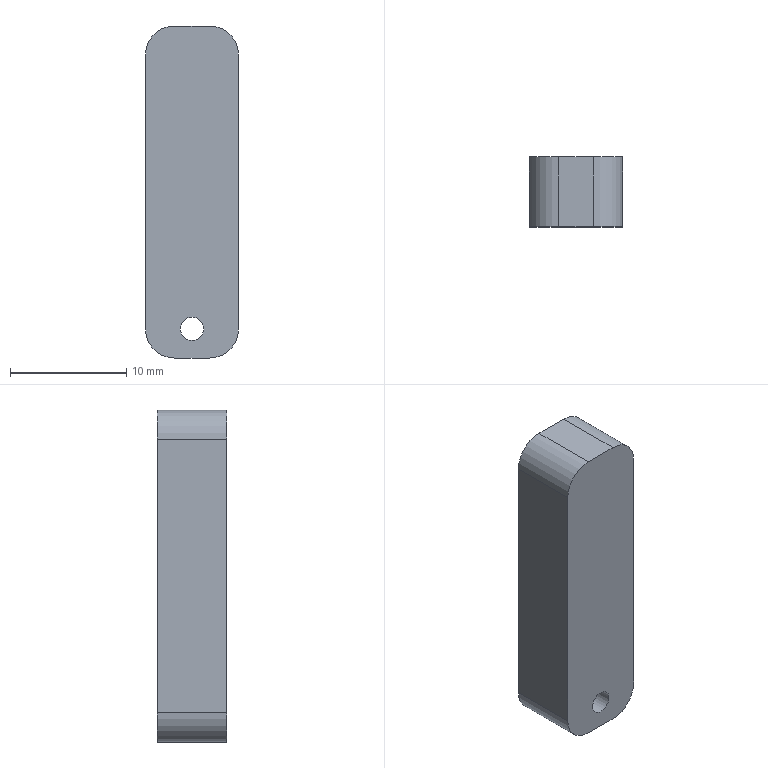Component | NX | ROBOT_ARM_SHORT_ARM | 1 solid | 11 faces | box 8 x 6 x 28.5 mm | volume 1317 mm3 | plane 6 | cylinder 5 | commonest cylinder face diameters 5 x4 2 x1
STEP:
#1=CARTESIAN_POINT('',(0.,0.,0.));
#2=DIRECTION('',(0.,0.,1.));
#3=DIRECTION('',(1.,0.,0.));
#4=AXIS2_PLACEMENT_3D('',#1,#2,#3);
#5=CARTESIAN_POINT('',(7.471,11.498,87.674));
#6=VERTEX_POINT('',#5);
#7=CARTESIAN_POINT('',(7.471,11.498,111.174));
#8=VERTEX_POINT('',#7);
#9=CARTESIAN_POINT('',(7.471,11.498,87.674));
#10=DIRECTION('',(0.,0.,1.));
#11=VECTOR('',#10,1.);
#12=LINE('',#9,#11);
#13=CARTESIAN_POINT('',(7.471,17.498,87.674));
#14=DIRECTION('',(1.,0.,-0.));
#15=DIRECTION('',(-0.,0.,-1.));
#16=AXIS2_PLACEMENT_3D('',#13,#14,#15);
#17=PLANE('',#16);
#18=CARTESIAN_POINT('',(0.,-6.));
#19=DIRECTION('',(-1.,0.));
#20=VECTOR('',#19,1.);
#21=LINE('',#18,#20);
#22=(GEOMETRIC_REPRESENTATION_CONTEXT(2)PARAMETRIC_REPRESENTATION_CONTEXT()REPRESENTATION_CONTEXT('',''));
#23=DEFINITIONAL_REPRESENTATION('',(#21),#22);
#24=PCURVE('',#17,#23);
#25=CARTESIAN_POINT('',(9.971,11.498,111.174));
#26=DIRECTION('',(0.,1.,0.));
#27=DIRECTION('',(1.,0.,0.));
#28=AXIS2_PLACEMENT_3D('',#25,#26,#27);
#29=PLANE('',#28);
#30=CARTESIAN_POINT('',(-2.5,23.5));
#31=DIRECTION('',(0.,-1.));
#32=VECTOR('',#31,1.);
#33=LINE('',#30,#32);
#34=(GEOMETRIC_REPRESENTATION_CONTEXT(2)PARAMETRIC_REPRESENTATION_CONTEXT()REPRESENTATION_CONTEXT('',''));
#35=DEFINITIONAL_REPRESENTATION('',(#33),#34);
#36=PCURVE('',#29,#35);
#37=SURFACE_CURVE('',#12,(#24,#36),.PCURVE_S1.);
#38=EDGE_CURVE('',#6,#8,#37,.T.);
#39=ORIENTED_EDGE('',*,*,#38,.T.);
#40=CARTESIAN_POINT('',(7.471,17.498,111.174));
#41=VERTEX_POINT('',#40);
#42=CARTESIAN_POINT('',(7.471,17.498,111.174));
#43=DIRECTION('',(0.,-1.,0.));
#44=VECTOR('',#43,1.);
#45=LINE('',#42,#44);
#46=CARTESIAN_POINT('',(-23.5,0.));
#47=DIRECTION('',(0.,-1.));
#48=VECTOR('',#47,1.);
#49=LINE('',#46,#48);
#50=(GEOMETRIC_REPRESENTATION_CONTEXT(2)PARAMETRIC_REPRESENTATION_CONTEXT()REPRESENTATION_CONTEXT('',''));
#51=DEFINITIONAL_REPRESENTATION('',(#49),#50);
#52=PCURVE('',#17,#51);
#53=CARTESIAN_POINT('',(9.971,17.498,111.174));
#54=DIRECTION('',(0.,-1.,0.));
#55=DIRECTION('',(-1.,0.,0.));
#56=AXIS2_PLACEMENT_3D('',#53,#54,#55);
#57=CYLINDRICAL_SURFACE('',#56,2.5);
#58=CARTESIAN_POINT('',(6.283,0.));
#59=DIRECTION('',(0.,1.));
#60=VECTOR('',#59,1.);
#61=LINE('',#58,#60);
#62=(GEOMETRIC_REPRESENTATION_CONTEXT(2)PARAMETRIC_REPRESENTATION_CONTEXT()REPRESENTATION_CONTEXT('',''));
#63=DEFINITIONAL_REPRESENTATION('',(#61),#62);
#64=PCURVE('',#57,#63);
#65=SURFACE_CURVE('',#45,(#52,#64),.PCURVE_S1.);
#66=EDGE_CURVE('',#41,#8,#65,.T.);
#67=ORIENTED_EDGE('',*,*,#66,.F.);
#68=CARTESIAN_POINT('',(7.471,17.498,87.674));
#69=VERTEX_POINT('',#68);
#70=CARTESIAN_POINT('',(7.471,17.498,87.674));
#71=DIRECTION('',(0.,0.,1.));
#72=VECTOR('',#71,1.);
#73=LINE('',#70,#72);
#74=CARTESIAN_POINT('',(0.,0.));
#75=DIRECTION('',(-1.,0.));
#76=VECTOR('',#75,1.);
#77=LINE('',#74,#76);
#78=(GEOMETRIC_REPRESENTATION_CONTEXT(2)PARAMETRIC_REPRESENTATION_CONTEXT()REPRESENTATION_CONTEXT('',''));
#79=DEFINITIONAL_REPRESENTATION('',(#77),#78);
#80=PCURVE('',#17,#79);
#81=CARTESIAN_POINT('',(9.971,17.498,111.174));
#82=DIRECTION('',(0.,1.,0.));
#83=DIRECTION('',(1.,0.,0.));
#84=AXIS2_PLACEMENT_3D('',#81,#82,#83);
#85=PLANE('',#84);
#86=CARTESIAN_POINT('',(-2.5,23.5));
#87=DIRECTION('',(0.,-1.));
#88=VECTOR('',#87,1.);
#89=LINE('',#86,#88);
#90=(GEOMETRIC_REPRESENTATION_CONTEXT(2)PARAMETRIC_REPRESENTATION_CONTEXT()REPRESENTATION_CONTEXT('',''));
#91=DEFINITIONAL_REPRESENTATION('',(#89),#90);
#92=PCURVE('',#85,#91);
#93=SURFACE_CURVE('',#73,(#80,#92),.PCURVE_S1.);
#94=EDGE_CURVE('',#69,#41,#93,.T.);
#95=ORIENTED_EDGE('',*,*,#94,.F.);
#96=CARTESIAN_POINT('',(7.471,17.498,87.674));
#97=DIRECTION('',(0.,-1.,0.));
#98=VECTOR('',#97,1.);
#99=LINE('',#96,#98);
#100=CARTESIAN_POINT('',(0.,0.));
#101=DIRECTION('',(0.,-1.));
#102=VECTOR('',#101,1.);
#103=LINE('',#100,#102);
#104=(GEOMETRIC_REPRESENTATION_CONTEXT(2)PARAMETRIC_REPRESENTATION_CONTEXT()REPRESENTATION_CONTEXT('',''));
#105=DEFINITIONAL_REPRESENTATION('',(#103),#104);
#106=PCURVE('',#17,#105);
#107=CARTESIAN_POINT('',(9.971,17.498,87.674));
#108=DIRECTION('',(0.,-1.,0.));
#109=DIRECTION('',(-1.,0.,0.));
#110=AXIS2_PLACEMENT_3D('',#107,#108,#109);
#111=CYLINDRICAL_SURFACE('',#110,2.5);
#112=CARTESIAN_POINT('',(0.,0.));
#113=DIRECTION('',(0.,1.));
#114=VECTOR('',#113,1.);
#115=LINE('',#112,#114);
#116=(GEOMETRIC_REPRESENTATION_CONTEXT(2)PARAMETRIC_REPRESENTATION_CONTEXT()REPRESENTATION_CONTEXT('',''));
#117=DEFINITIONAL_REPRESENTATION('',(#115),#116);
#118=PCURVE('',#111,#117);
#119=SURFACE_CURVE('',#99,(#106,#118),.PCURVE_S1.);
#120=EDGE_CURVE('',#69,#6,#119,.T.);
#121=ORIENTED_EDGE('',*,*,#120,.T.);
#122=EDGE_LOOP('',(#39,#67,#95,#121));
#123=FACE_BOUND('',#122,.T.);
#124=ADVANCED_FACE('',(#123),#17,.F.);
#125=CARTESIAN_POINT('',(9.971,11.498,113.674));
#126=VERTEX_POINT('',#125);
#127=CARTESIAN_POINT('',(9.971,11.498,111.174));
#128=DIRECTION('',(0.,1.,0.));
#129=DIRECTION('',(1.,0.,0.));
#130=AXIS2_PLACEMENT_3D('',#127,#128,#129);
#131=CIRCLE('',#130,2.5);
#132=CARTESIAN_POINT('',(9.425,6.));
#133=DIRECTION('',(-1.,0.));
#134=VECTOR('',#133,1.);
#135=LINE('',#132,#134);
#136=(GEOMETRIC_REPRESENTATION_CONTEXT(2)PARAMETRIC_REPRESENTATION_CONTEXT()REPRESENTATION_CONTEXT('',''));
#137=DEFINITIONAL_REPRESENTATION('',(#135),#136);
#138=PCURVE('',#57,#137);
#139=CARTESIAN_POINT('',(0.,0.));
#140=DIRECTION('',(1.,0.));
#141=AXIS2_PLACEMENT_2D('',#139,#140);
#142=CIRCLE('',#141,2.5);
#143=(GEOMETRIC_REPRESENTATION_CONTEXT(2)PARAMETRIC_REPRESENTATION_CONTEXT()REPRESENTATION_CONTEXT('',''));
#144=DEFINITIONAL_REPRESENTATION('',(#142),#143);
#145=PCURVE('',#29,#144);
#146=SURFACE_CURVE('',#131,(#138,#145),.PCURVE_S1.);
#147=EDGE_CURVE('',#8,#126,#146,.T.);
#148=ORIENTED_EDGE('',*,*,#147,.T.);
#149=CARTESIAN_POINT('',(9.971,17.498,113.674));
#150=VERTEX_POINT('',#149);
#151=CARTESIAN_POINT('',(9.971,17.498,113.674));
#152=DIRECTION('',(0.,-1.,0.));
#153=VECTOR('',#152,1.);
#154=LINE('',#151,#153);
#155=CARTESIAN_POINT('',(4.712,0.));
#156=DIRECTION('',(0.,1.));
#157=VECTOR('',#156,1.);
#158=LINE('',#155,#157);
#159=(GEOMETRIC_REPRESENTATION_CONTEXT(2)PARAMETRIC_REPRESENTATION_CONTEXT()REPRESENTATION_CONTEXT('',''));
#160=DEFINITIONAL_REPRESENTATION('',(#158),#159);
#161=PCURVE('',#57,#160);
#162=CARTESIAN_POINT('',(9.971,17.498,113.674));
#163=DIRECTION('',(-0.,0.,-1.));
#164=DIRECTION('',(-1.,0.,0.));
#165=AXIS2_PLACEMENT_3D('',#162,#163,#164);
#166=PLANE('',#165);
#167=CARTESIAN_POINT('',(0.,0.));
#168=DIRECTION('',(0.,-1.));
#169=VECTOR('',#168,1.);
#170=LINE('',#167,#169);
#171=(GEOMETRIC_REPRESENTATION_CONTEXT(2)PARAMETRIC_REPRESENTATION_CONTEXT()REPRESENTATION_CONTEXT('',''));
#172=DEFINITIONAL_REPRESENTATION('',(#170),#171);
#173=PCURVE('',#166,#172);
#174=SURFACE_CURVE('',#154,(#161,#173),.PCURVE_S1.);
#175=EDGE_CURVE('',#150,#126,#174,.T.);
#176=ORIENTED_EDGE('',*,*,#175,.F.);
#177=CARTESIAN_POINT('',(9.971,17.498,111.174));
#178=DIRECTION('',(0.,1.,0.));
#179=DIRECTION('',(1.,0.,0.));
#180=AXIS2_PLACEMENT_3D('',#177,#178,#179);
#181=CIRCLE('',#180,2.5);
#182=CARTESIAN_POINT('',(9.425,0.));
#183=DIRECTION('',(-1.,0.));
#184=VECTOR('',#183,1.);
#185=LINE('',#182,#184);
#186=(GEOMETRIC_REPRESENTATION_CONTEXT(2)PARAMETRIC_REPRESENTATION_CONTEXT()REPRESENTATION_CONTEXT('',''));
#187=DEFINITIONAL_REPRESENTATION('',(#185),#186);
#188=PCURVE('',#57,#187);
#189=CARTESIAN_POINT('',(0.,0.));
#190=DIRECTION('',(1.,0.));
#191=AXIS2_PLACEMENT_2D('',#189,#190);
#192=CIRCLE('',#191,2.5);
#193=(GEOMETRIC_REPRESENTATION_CONTEXT(2)PARAMETRIC_REPRESENTATION_CONTEXT()REPRESENTATION_CONTEXT('',''));
#194=DEFINITIONAL_REPRESENTATION('',(#192),#193);
#195=PCURVE('',#85,#194);
#196=SURFACE_CURVE('',#181,(#188,#195),.PCURVE_S1.);
#197=EDGE_CURVE('',#41,#150,#196,.T.);
#198=ORIENTED_EDGE('',*,*,#197,.F.);
#199=ORIENTED_EDGE('',*,*,#66,.T.);
#200=EDGE_LOOP('',(#148,#176,#198,#199));
#201=FACE_BOUND('',#200,.T.);
#202=ADVANCED_FACE('',(#201),#57,.T.);
#203=CARTESIAN_POINT('',(12.971,11.498,113.674));
#204=VERTEX_POINT('',#203);
#205=CARTESIAN_POINT('',(9.971,11.498,113.674));
#206=DIRECTION('',(1.,0.,-0.));
#207=VECTOR('',#206,1.);
#208=LINE('',#205,#207);
#209=CARTESIAN_POINT('',(0.,-6.));
#210=DIRECTION('',(-1.,0.));
#211=VECTOR('',#210,1.);
#212=LINE('',#209,#211);
#213=(GEOMETRIC_REPRESENTATION_CONTEXT(2)PARAMETRIC_REPRESENTATION_CONTEXT()REPRESENTATION_CONTEXT('',''));
#214=DEFINITIONAL_REPRESENTATION('',(#212),#213);
#215=PCURVE('',#166,#214);
#216=CARTESIAN_POINT('',(0.,-2.5));
#217=DIRECTION('',(1.,0.));
#218=VECTOR('',#217,1.);
#219=LINE('',#216,#218);
#220=(GEOMETRIC_REPRESENTATION_CONTEXT(2)PARAMETRIC_REPRESENTATION_CONTEXT()REPRESENTATION_CONTEXT('',''));
#221=DEFINITIONAL_REPRESENTATION('',(#219),#220);
#222=PCURVE('',#29,#221);
#223=SURFACE_CURVE('',#208,(#215,#222),.PCURVE_S1.);
#224=EDGE_CURVE('',#126,#204,#223,.T.);
#225=ORIENTED_EDGE('',*,*,#224,.T.);
#226=CARTESIAN_POINT('',(12.971,17.498,113.674));
#227=VERTEX_POINT('',#226);
#228=CARTESIAN_POINT('',(12.971,17.498,113.674));
#229=DIRECTION('',(0.,-1.,0.));
#230=VECTOR('',#229,1.);
#231=LINE('',#228,#230);
#232=CARTESIAN_POINT('',(-3.,0.));
#233=DIRECTION('',(0.,-1.));
#234=VECTOR('',#233,1.);
#235=LINE('',#232,#234);
#236=(GEOMETRIC_REPRESENTATION_CONTEXT(2)PARAMETRIC_REPRESENTATION_CONTEXT()REPRESENTATION_CONTEXT('',''));
#237=DEFINITIONAL_REPRESENTATION('',(#235),#236);
#238=PCURVE('',#166,#237);
#239=CARTESIAN_POINT('',(12.971,17.498,111.174));
#240=DIRECTION('',(0.,-1.,0.));
#241=DIRECTION('',(-1.,0.,0.));
#242=AXIS2_PLACEMENT_3D('',#239,#240,#241);
#243=CYLINDRICAL_SURFACE('',#242,2.5);
#244=CARTESIAN_POINT('',(4.712,0.));
#245=DIRECTION('',(0.,1.));
#246=VECTOR('',#245,1.);
#247=LINE('',#244,#246);
#248=(GEOMETRIC_REPRESENTATION_CONTEXT(2)PARAMETRIC_REPRESENTATION_CONTEXT()REPRESENTATION_CONTEXT('',''));
#249=DEFINITIONAL_REPRESENTATION('',(#247),#248);
#250=PCURVE('',#243,#249);
#251=SURFACE_CURVE('',#231,(#238,#250),.PCURVE_S1.);
#252=EDGE_CURVE('',#227,#204,#251,.T.);
#253=ORIENTED_EDGE('',*,*,#252,.F.);
#254=CARTESIAN_POINT('',(9.971,17.498,113.674));
#255=DIRECTION('',(1.,0.,-0.));
#256=VECTOR('',#255,1.);
#257=LINE('',#254,#256);
#258=CARTESIAN_POINT('',(0.,0.));
#259=DIRECTION('',(-1.,0.));
#260=VECTOR('',#259,1.);
#261=LINE('',#258,#260);
#262=(GEOMETRIC_REPRESENTATION_CONTEXT(2)PARAMETRIC_REPRESENTATION_CONTEXT()REPRESENTATION_CONTEXT('',''));
#263=DEFINITIONAL_REPRESENTATION('',(#261),#262);
#264=PCURVE('',#166,#263);
#265=CARTESIAN_POINT('',(0.,-2.5));
#266=DIRECTION('',(1.,0.));
#267=VECTOR('',#266,1.);
#268=LINE('',#265,#267);
#269=(GEOMETRIC_REPRESENTATION_CONTEXT(2)PARAMETRIC_REPRESENTATION_CONTEXT()REPRESENTATION_CONTEXT('',''));
#270=DEFINITIONAL_REPRESENTATION('',(#268),#269);
#271=PCURVE('',#85,#270);
#272=SURFACE_CURVE('',#257,(#264,#271),.PCURVE_S1.);
#273=EDGE_CURVE('',#150,#227,#272,.T.);
#274=ORIENTED_EDGE('',*,*,#273,.F.);
#275=ORIENTED_EDGE('',*,*,#175,.T.);
#276=EDGE_LOOP('',(#225,#253,#274,#275));
#277=FACE_BOUND('',#276,.T.);
#278=ADVANCED_FACE('',(#277),#166,.F.);
#279=CARTESIAN_POINT('',(15.471,11.498,111.174));
#280=VERTEX_POINT('',#279);
#281=CARTESIAN_POINT('',(12.971,11.498,111.174));
#282=DIRECTION('',(0.,1.,0.));
#283=DIRECTION('',(1.,0.,0.));
#284=AXIS2_PLACEMENT_3D('',#281,#282,#283);
#285=CIRCLE('',#284,2.5);
#286=CARTESIAN_POINT('',(9.425,6.));
#287=DIRECTION('',(-1.,0.));
#288=VECTOR('',#287,1.);
#289=LINE('',#286,#288);
#290=(GEOMETRIC_REPRESENTATION_CONTEXT(2)PARAMETRIC_REPRESENTATION_CONTEXT()REPRESENTATION_CONTEXT('',''));
#291=DEFINITIONAL_REPRESENTATION('',(#289),#290);
#292=PCURVE('',#243,#291);
#293=CARTESIAN_POINT('',(3.,0.));
#294=DIRECTION('',(1.,0.));
#295=AXIS2_PLACEMENT_2D('',#293,#294);
#296=CIRCLE('',#295,2.5);
#297=(GEOMETRIC_REPRESENTATION_CONTEXT(2)PARAMETRIC_REPRESENTATION_CONTEXT()REPRESENTATION_CONTEXT('',''));
#298=DEFINITIONAL_REPRESENTATION('',(#296),#297);
#299=PCURVE('',#29,#298);
#300=SURFACE_CURVE('',#285,(#292,#299),.PCURVE_S1.);
#301=EDGE_CURVE('',#204,#280,#300,.T.);
#302=ORIENTED_EDGE('',*,*,#301,.T.);
#303=CARTESIAN_POINT('',(15.471,17.498,111.174));
#304=VERTEX_POINT('',#303);
#305=CARTESIAN_POINT('',(15.471,17.498,111.174));
#306=DIRECTION('',(0.,-1.,0.));
#307=VECTOR('',#306,1.);
#308=LINE('',#305,#307);
#309=CARTESIAN_POINT('',(3.142,0.));
#310=DIRECTION('',(0.,1.));
#311=VECTOR('',#310,1.);
#312=LINE('',#309,#311);
#313=(GEOMETRIC_REPRESENTATION_CONTEXT(2)PARAMETRIC_REPRESENTATION_CONTEXT()REPRESENTATION_CONTEXT('',''));
#314=DEFINITIONAL_REPRESENTATION('',(#312),#313);
#315=PCURVE('',#243,#314);
#316=CARTESIAN_POINT('',(15.471,17.498,111.174));
#317=DIRECTION('',(-1.,0.,0.));
#318=DIRECTION('',(0.,0.,1.));
#319=AXIS2_PLACEMENT_3D('',#316,#317,#318);
#320=PLANE('',#319);
#321=CARTESIAN_POINT('',(0.,0.));
#322=DIRECTION('',(0.,-1.));
#323=VECTOR('',#322,1.);
#324=LINE('',#321,#323);
#325=(GEOMETRIC_REPRESENTATION_CONTEXT(2)PARAMETRIC_REPRESENTATION_CONTEXT()REPRESENTATION_CONTEXT('',''));
#326=DEFINITIONAL_REPRESENTATION('',(#324),#325);
#327=PCURVE('',#320,#326);
#328=SURFACE_CURVE('',#308,(#315,#327),.PCURVE_S1.);
#329=EDGE_CURVE('',#304,#280,#328,.T.);
#330=ORIENTED_EDGE('',*,*,#329,.F.);
#331=CARTESIAN_POINT('',(12.971,17.498,111.174));
#332=DIRECTION('',(0.,1.,0.));
#333=DIRECTION('',(1.,0.,0.));
#334=AXIS2_PLACEMENT_3D('',#331,#332,#333);
#335=CIRCLE('',#334,2.5);
#336=CARTESIAN_POINT('',(9.425,0.));
#337=DIRECTION('',(-1.,0.));
#338=VECTOR('',#337,1.);
#339=LINE('',#336,#338);
#340=(GEOMETRIC_REPRESENTATION_CONTEXT(2)PARAMETRIC_REPRESENTATION_CONTEXT()REPRESENTATION_CONTEXT('',''));
#341=DEFINITIONAL_REPRESENTATION('',(#339),#340);
#342=PCURVE('',#243,#341);
#343=CARTESIAN_POINT('',(3.,0.));
#344=DIRECTION('',(1.,0.));
#345=AXIS2_PLACEMENT_2D('',#343,#344);
#346=CIRCLE('',#345,2.5);
#347=(GEOMETRIC_REPRESENTATION_CONTEXT(2)PARAMETRIC_REPRESENTATION_CONTEXT()REPRESENTATION_CONTEXT('',''));
#348=DEFINITIONAL_REPRESENTATION('',(#346),#347);
#349=PCURVE('',#85,#348);
#350=SURFACE_CURVE('',#335,(#342,#349),.PCURVE_S1.);
#351=EDGE_CURVE('',#227,#304,#350,.T.);
#352=ORIENTED_EDGE('',*,*,#351,.F.);
#353=ORIENTED_EDGE('',*,*,#252,.T.);
#354=EDGE_LOOP('',(#302,#330,#352,#353));
#355=FACE_BOUND('',#354,.T.);
#356=ADVANCED_FACE('',(#355),#243,.T.);
#357=CARTESIAN_POINT('',(15.471,11.498,87.674));
#358=VERTEX_POINT('',#357);
#359=CARTESIAN_POINT('',(15.471,11.498,111.174));
#360=DIRECTION('',(-0.,0.,-1.));
#361=VECTOR('',#360,1.);
#362=LINE('',#359,#361);
#363=CARTESIAN_POINT('',(0.,-6.));
#364=DIRECTION('',(-1.,0.));
#365=VECTOR('',#364,1.);
#366=LINE('',#363,#365);
#367=(GEOMETRIC_REPRESENTATION_CONTEXT(2)PARAMETRIC_REPRESENTATION_CONTEXT()REPRESENTATION_CONTEXT('',''));
#368=DEFINITIONAL_REPRESENTATION('',(#366),#367);
#369=PCURVE('',#320,#368);
#370=CARTESIAN_POINT('',(5.5,0.));
#371=DIRECTION('',(-0.,1.));
#372=VECTOR('',#371,1.);
#373=LINE('',#370,#372);
#374=(GEOMETRIC_REPRESENTATION_CONTEXT(2)PARAMETRIC_REPRESENTATION_CONTEXT()REPRESENTATION_CONTEXT('',''));
#375=DEFINITIONAL_REPRESENTATION('',(#373),#374);
#376=PCURVE('',#29,#375);
#377=SURFACE_CURVE('',#362,(#369,#376),.PCURVE_S1.);
#378=EDGE_CURVE('',#280,#358,#377,.T.);
#379=ORIENTED_EDGE('',*,*,#378,.T.);
#380=CARTESIAN_POINT('',(15.471,17.498,87.674));
#381=VERTEX_POINT('',#380);
#382=CARTESIAN_POINT('',(15.471,17.498,87.674));
#383=DIRECTION('',(0.,-1.,0.));
#384=VECTOR('',#383,1.);
#385=LINE('',#382,#384);
#386=CARTESIAN_POINT('',(-23.5,0.));
#387=DIRECTION('',(0.,-1.));
#388=VECTOR('',#387,1.);
#389=LINE('',#386,#388);
#390=(GEOMETRIC_REPRESENTATION_CONTEXT(2)PARAMETRIC_REPRESENTATION_CONTEXT()REPRESENTATION_CONTEXT('',''));
#391=DEFINITIONAL_REPRESENTATION('',(#389),#390);
#392=PCURVE('',#320,#391);
#393=CARTESIAN_POINT('',(12.971,17.498,87.674));
#394=DIRECTION('',(0.,-1.,0.));
#395=DIRECTION('',(-1.,0.,0.));
#396=AXIS2_PLACEMENT_3D('',#393,#394,#395);
#397=CYLINDRICAL_SURFACE('',#396,2.5);
#398=CARTESIAN_POINT('',(3.142,0.));
#399=DIRECTION('',(0.,1.));
#400=VECTOR('',#399,1.);
#401=LINE('',#398,#400);
#402=(GEOMETRIC_REPRESENTATION_CONTEXT(2)PARAMETRIC_REPRESENTATION_CONTEXT()REPRESENTATION_CONTEXT('',''));
#403=DEFINITIONAL_REPRESENTATION('',(#401),#402);
#404=PCURVE('',#397,#403);
#405=SURFACE_CURVE('',#385,(#392,#404),.PCURVE_S1.);
#406=EDGE_CURVE('',#381,#358,#405,.T.);
#407=ORIENTED_EDGE('',*,*,#406,.F.);
#408=CARTESIAN_POINT('',(15.471,17.498,111.174));
#409=DIRECTION('',(-0.,0.,-1.));
#410=VECTOR('',#409,1.);
#411=LINE('',#408,#410);
#412=CARTESIAN_POINT('',(0.,0.));
#413=DIRECTION('',(-1.,0.));
#414=VECTOR('',#413,1.);
#415=LINE('',#412,#414);
#416=(GEOMETRIC_REPRESENTATION_CONTEXT(2)PARAMETRIC_REPRESENTATION_CONTEXT()REPRESENTATION_CONTEXT('',''));
#417=DEFINITIONAL_REPRESENTATION('',(#415),#416);
#418=PCURVE('',#320,#417);
#419=CARTESIAN_POINT('',(5.5,0.));
#420=DIRECTION('',(-0.,1.));
#421=VECTOR('',#420,1.);
#422=LINE('',#419,#421);
#423=(GEOMETRIC_REPRESENTATION_CONTEXT(2)PARAMETRIC_REPRESENTATION_CONTEXT()REPRESENTATION_CONTEXT('',''));
#424=DEFINITIONAL_REPRESENTATION('',(#422),#423);
#425=PCURVE('',#85,#424);
#426=SURFACE_CURVE('',#411,(#418,#425),.PCURVE_S1.);
#427=EDGE_CURVE('',#304,#381,#426,.T.);
#428=ORIENTED_EDGE('',*,*,#427,.F.);
#429=ORIENTED_EDGE('',*,*,#329,.T.);
#430=EDGE_LOOP('',(#379,#407,#428,#429));
#431=FACE_BOUND('',#430,.T.);
#432=ADVANCED_FACE('',(#431),#320,.F.);
#433=CARTESIAN_POINT('',(12.971,11.498,85.174));
#434=VERTEX_POINT('',#433);
#435=CARTESIAN_POINT('',(12.971,11.498,87.674));
#436=DIRECTION('',(0.,1.,0.));
#437=DIRECTION('',(1.,0.,0.));
#438=AXIS2_PLACEMENT_3D('',#435,#436,#437);
#439=CIRCLE('',#438,2.5);
#440=CARTESIAN_POINT('',(3.142,6.));
#441=DIRECTION('',(-1.,0.));
#442=VECTOR('',#441,1.);
#443=LINE('',#440,#442);
#444=(GEOMETRIC_REPRESENTATION_CONTEXT(2)PARAMETRIC_REPRESENTATION_CONTEXT()REPRESENTATION_CONTEXT('',''));
#445=DEFINITIONAL_REPRESENTATION('',(#443),#444);
#446=PCURVE('',#397,#445);
#447=CARTESIAN_POINT('',(3.,23.5));
#448=DIRECTION('',(1.,0.));
#449=AXIS2_PLACEMENT_2D('',#447,#448);
#450=CIRCLE('',#449,2.5);
#451=(GEOMETRIC_REPRESENTATION_CONTEXT(2)PARAMETRIC_REPRESENTATION_CONTEXT()REPRESENTATION_CONTEXT('',''));
#452=DEFINITIONAL_REPRESENTATION('',(#450),#451);
#453=PCURVE('',#29,#452);
#454=SURFACE_CURVE('',#439,(#446,#453),.PCURVE_S1.);
#455=EDGE_CURVE('',#358,#434,#454,.T.);
#456=ORIENTED_EDGE('',*,*,#455,.T.);
#457=CARTESIAN_POINT('',(12.971,17.498,85.174));
#458=VERTEX_POINT('',#457);
#459=CARTESIAN_POINT('',(12.971,17.498,85.174));
#460=DIRECTION('',(0.,-1.,0.));
#461=VECTOR('',#460,1.);
#462=LINE('',#459,#461);
#463=CARTESIAN_POINT('',(1.571,0.));
#464=DIRECTION('',(0.,1.));
#465=VECTOR('',#464,1.);
#466=LINE('',#463,#465);
#467=(GEOMETRIC_REPRESENTATION_CONTEXT(2)PARAMETRIC_REPRESENTATION_CONTEXT()REPRESENTATION_CONTEXT('',''));
#468=DEFINITIONAL_REPRESENTATION('',(#466),#467);
#469=PCURVE('',#397,#468);
#470=CARTESIAN_POINT('',(12.971,17.498,85.174));
#471=DIRECTION('',(0.,0.,1.));
#472=DIRECTION('',(0.,-1.,0.));
#473=AXIS2_PLACEMENT_3D('',#470,#471,#472);
#474=PLANE('',#473);
#475=CARTESIAN_POINT('',(0.,0.));
#476=DIRECTION('',(1.,0.));
#477=VECTOR('',#476,1.);
#478=LINE('',#475,#477);
#479=(GEOMETRIC_REPRESENTATION_CONTEXT(2)PARAMETRIC_REPRESENTATION_CONTEXT()REPRESENTATION_CONTEXT('',''));
#480=DEFINITIONAL_REPRESENTATION('',(#478),#479);
#481=PCURVE('',#474,#480);
#482=SURFACE_CURVE('',#462,(#469,#481),.PCURVE_S1.);
#483=EDGE_CURVE('',#458,#434,#482,.T.);
#484=ORIENTED_EDGE('',*,*,#483,.F.);
#485=CARTESIAN_POINT('',(12.971,17.498,87.674));
#486=DIRECTION('',(0.,1.,0.));
#487=DIRECTION('',(1.,0.,0.));
#488=AXIS2_PLACEMENT_3D('',#485,#486,#487);
#489=CIRCLE('',#488,2.5);
#490=CARTESIAN_POINT('',(3.142,0.));
#491=DIRECTION('',(-1.,0.));
#492=VECTOR('',#491,1.);
#493=LINE('',#490,#492);
#494=(GEOMETRIC_REPRESENTATION_CONTEXT(2)PARAMETRIC_REPRESENTATION_CONTEXT()REPRESENTATION_CONTEXT('',''));
#495=DEFINITIONAL_REPRESENTATION('',(#493),#494);
#496=PCURVE('',#397,#495);
#497=CARTESIAN_POINT('',(3.,23.5));
#498=DIRECTION('',(1.,0.));
#499=AXIS2_PLACEMENT_2D('',#497,#498);
#500=CIRCLE('',#499,2.5);
#501=(GEOMETRIC_REPRESENTATION_CONTEXT(2)PARAMETRIC_REPRESENTATION_CONTEXT()REPRESENTATION_CONTEXT('',''));
#502=DEFINITIONAL_REPRESENTATION('',(#500),#501);
#503=PCURVE('',#85,#502);
#504=SURFACE_CURVE('',#489,(#496,#503),.PCURVE_S1.);
#505=EDGE_CURVE('',#381,#458,#504,.T.);
#506=ORIENTED_EDGE('',*,*,#505,.F.);
#507=ORIENTED_EDGE('',*,*,#406,.T.);
#508=EDGE_LOOP('',(#456,#484,#506,#507));
#509=FACE_BOUND('',#508,.T.);
#510=ADVANCED_FACE('',(#509),#397,.T.);
#511=CARTESIAN_POINT('',(9.971,11.498,85.174));
#512=VERTEX_POINT('',#511);
#513=CARTESIAN_POINT('',(12.971,11.498,85.174));
#514=DIRECTION('',(-1.,0.,0.));
#515=VECTOR('',#514,1.);
#516=LINE('',#513,#515);
#517=CARTESIAN_POINT('',(6.,0.));
#518=DIRECTION('',(0.,-1.));
#519=VECTOR('',#518,1.);
#520=LINE('',#517,#519);
#521=(GEOMETRIC_REPRESENTATION_CONTEXT(2)PARAMETRIC_REPRESENTATION_CONTEXT()REPRESENTATION_CONTEXT('',''));
#522=DEFINITIONAL_REPRESENTATION('',(#520),#521);
#523=PCURVE('',#474,#522);
#524=CARTESIAN_POINT('',(3.,26.));
#525=DIRECTION('',(-1.,0.));
#526=VECTOR('',#525,1.);
#527=LINE('',#524,#526);
#528=(GEOMETRIC_REPRESENTATION_CONTEXT(2)PARAMETRIC_REPRESENTATION_CONTEXT()REPRESENTATION_CONTEXT('',''));
#529=DEFINITIONAL_REPRESENTATION('',(#527),#528);
#530=PCURVE('',#29,#529);
#531=SURFACE_CURVE('',#516,(#523,#530),.PCURVE_S1.);
#532=EDGE_CURVE('',#434,#512,#531,.T.);
#533=ORIENTED_EDGE('',*,*,#532,.T.);
#534=CARTESIAN_POINT('',(9.971,17.498,85.174));
#535=VERTEX_POINT('',#534);
#536=CARTESIAN_POINT('',(9.971,17.498,85.174));
#537=DIRECTION('',(0.,-1.,0.));
#538=VECTOR('',#537,1.);
#539=LINE('',#536,#538);
#540=CARTESIAN_POINT('',(0.,-3.));
#541=DIRECTION('',(1.,0.));
#542=VECTOR('',#541,1.);
#543=LINE('',#540,#542);
#544=(GEOMETRIC_REPRESENTATION_CONTEXT(2)PARAMETRIC_REPRESENTATION_CONTEXT()REPRESENTATION_CONTEXT('',''));
#545=DEFINITIONAL_REPRESENTATION('',(#543),#544);
#546=PCURVE('',#474,#545);
#547=CARTESIAN_POINT('',(1.571,0.));
#548=DIRECTION('',(0.,1.));
#549=VECTOR('',#548,1.);
#550=LINE('',#547,#549);
#551=(GEOMETRIC_REPRESENTATION_CONTEXT(2)PARAMETRIC_REPRESENTATION_CONTEXT()REPRESENTATION_CONTEXT('',''));
#552=DEFINITIONAL_REPRESENTATION('',(#550),#551);
#553=PCURVE('',#111,#552);
#554=SURFACE_CURVE('',#539,(#546,#553),.PCURVE_S1.);
#555=EDGE_CURVE('',#535,#512,#554,.T.);
#556=ORIENTED_EDGE('',*,*,#555,.F.);
#557=CARTESIAN_POINT('',(12.971,17.498,85.174));
#558=DIRECTION('',(-1.,0.,0.));
#559=VECTOR('',#558,1.);
#560=LINE('',#557,#559);
#561=CARTESIAN_POINT('',(0.,0.));
#562=DIRECTION('',(0.,-1.));
#563=VECTOR('',#562,1.);
#564=LINE('',#561,#563);
#565=(GEOMETRIC_REPRESENTATION_CONTEXT(2)PARAMETRIC_REPRESENTATION_CONTEXT()REPRESENTATION_CONTEXT('',''));
#566=DEFINITIONAL_REPRESENTATION('',(#564),#565);
#567=PCURVE('',#474,#566);
#568=CARTESIAN_POINT('',(3.,26.));
#569=DIRECTION('',(-1.,0.));
#570=VECTOR('',#569,1.);
#571=LINE('',#568,#570);
#572=(GEOMETRIC_REPRESENTATION_CONTEXT(2)PARAMETRIC_REPRESENTATION_CONTEXT()REPRESENTATION_CONTEXT('',''));
#573=DEFINITIONAL_REPRESENTATION('',(#571),#572);
#574=PCURVE('',#85,#573);
#575=SURFACE_CURVE('',#560,(#567,#574),.PCURVE_S1.);
#576=EDGE_CURVE('',#458,#535,#575,.T.);
#577=ORIENTED_EDGE('',*,*,#576,.F.);
#578=ORIENTED_EDGE('',*,*,#483,.T.);
#579=EDGE_LOOP('',(#533,#556,#577,#578));
#580=FACE_BOUND('',#579,.T.);
#581=ADVANCED_FACE('',(#580),#474,.F.);
#582=CARTESIAN_POINT('',(9.971,11.498,87.674));
#583=DIRECTION('',(0.,1.,0.));
#584=DIRECTION('',(1.,0.,0.));
#585=AXIS2_PLACEMENT_3D('',#582,#583,#584);
#586=CIRCLE('',#585,2.5);
#587=CARTESIAN_POINT('',(3.142,6.));
#588=DIRECTION('',(-1.,0.));
#589=VECTOR('',#588,1.);
#590=LINE('',#587,#589);
#591=(GEOMETRIC_REPRESENTATION_CONTEXT(2)PARAMETRIC_REPRESENTATION_CONTEXT()REPRESENTATION_CONTEXT('',''));
#592=DEFINITIONAL_REPRESENTATION('',(#590),#591);
#593=PCURVE('',#111,#592);
#594=CARTESIAN_POINT('',(0.,23.5));
#595=DIRECTION('',(1.,0.));
#596=AXIS2_PLACEMENT_2D('',#594,#595);
#597=CIRCLE('',#596,2.5);
#598=(GEOMETRIC_REPRESENTATION_CONTEXT(2)PARAMETRIC_REPRESENTATION_CONTEXT()REPRESENTATION_CONTEXT('',''));
#599=DEFINITIONAL_REPRESENTATION('',(#597),#598);
#600=PCURVE('',#29,#599);
#601=SURFACE_CURVE('',#586,(#593,#600),.PCURVE_S1.);
#602=EDGE_CURVE('',#512,#6,#601,.T.);
#603=ORIENTED_EDGE('',*,*,#602,.T.);
#604=ORIENTED_EDGE('',*,*,#120,.F.);
#605=CARTESIAN_POINT('',(9.971,17.498,87.674));
#606=DIRECTION('',(0.,1.,0.));
#607=DIRECTION('',(1.,0.,0.));
#608=AXIS2_PLACEMENT_3D('',#605,#606,#607);
#609=CIRCLE('',#608,2.5);
#610=CARTESIAN_POINT('',(3.142,0.));
#611=DIRECTION('',(-1.,0.));
#612=VECTOR('',#611,1.);
#613=LINE('',#610,#612);
#614=(GEOMETRIC_REPRESENTATION_CONTEXT(2)PARAMETRIC_REPRESENTATION_CONTEXT()REPRESENTATION_CONTEXT('',''));
#615=DEFINITIONAL_REPRESENTATION('',(#613),#614);
#616=PCURVE('',#111,#615);
#617=CARTESIAN_POINT('',(0.,23.5));
#618=DIRECTION('',(1.,0.));
#619=AXIS2_PLACEMENT_2D('',#617,#618);
#620=CIRCLE('',#619,2.5);
#621=(GEOMETRIC_REPRESENTATION_CONTEXT(2)PARAMETRIC_REPRESENTATION_CONTEXT()REPRESENTATION_CONTEXT('',''));
#622=DEFINITIONAL_REPRESENTATION('',(#620),#621);
#623=PCURVE('',#85,#622);
#624=SURFACE_CURVE('',#609,(#616,#623),.PCURVE_S1.);
#625=EDGE_CURVE('',#535,#69,#624,.T.);
#626=ORIENTED_EDGE('',*,*,#625,.F.);
#627=ORIENTED_EDGE('',*,*,#555,.T.);
#628=EDGE_LOOP('',(#603,#604,#626,#627));
#629=FACE_BOUND('',#628,.T.);
#630=ADVANCED_FACE('',(#629),#111,.T.);
#631=CARTESIAN_POINT('',(12.471,17.498,87.674));
#632=VERTEX_POINT('',#631);
#633=CARTESIAN_POINT('',(11.471,17.498,87.674));
#634=DIRECTION('',(0.,1.,0.));
#635=DIRECTION('',(1.,0.,0.));
#636=AXIS2_PLACEMENT_3D('',#633,#634,#635);
#637=CIRCLE('',#636,1.);
#638=CARTESIAN_POINT('',(11.471,17.498,87.674));
#639=DIRECTION('',(0.,-1.,0.));
#640=DIRECTION('',(-1.,0.,0.));
#641=AXIS2_PLACEMENT_3D('',#638,#639,#640);
#642=CYLINDRICAL_SURFACE('',#641,1.);
#643=CARTESIAN_POINT('',(9.425,0.));
#644=DIRECTION('',(-1.,0.));
#645=VECTOR('',#644,1.);
#646=LINE('',#643,#645);
#647=(GEOMETRIC_REPRESENTATION_CONTEXT(2)PARAMETRIC_REPRESENTATION_CONTEXT()REPRESENTATION_CONTEXT('',''));
#648=DEFINITIONAL_REPRESENTATION('',(#646),#647);
#649=PCURVE('',#642,#648);
#650=CARTESIAN_POINT('',(1.5,23.5));
#651=DIRECTION('',(1.,0.));
#652=AXIS2_PLACEMENT_2D('',#650,#651);
#653=CIRCLE('',#652,1.);
#654=(GEOMETRIC_REPRESENTATION_CONTEXT(2)PARAMETRIC_REPRESENTATION_CONTEXT()REPRESENTATION_CONTEXT('',''));
#655=DEFINITIONAL_REPRESENTATION('',(#653),#654);
#656=PCURVE('',#85,#655);
#657=SURFACE_CURVE('',#637,(#649,#656),.PCURVE_S1.);
#658=EDGE_CURVE('',#632,#632,#657,.T.);
#659=ORIENTED_EDGE('',*,*,#658,.F.);
#660=CARTESIAN_POINT('',(12.471,11.498,87.674));
#661=VERTEX_POINT('',#660);
#662=CARTESIAN_POINT('',(12.471,17.498,87.674));
#663=CARTESIAN_POINT('',(12.471,11.498,87.674));
#664=B_SPLINE_CURVE_WITH_KNOTS('',1,(#662,#663),.UNSPECIFIED.,.F.,.F.,(2,2),(0.,6.),.PIECEWISE_BEZIER_KNOTS.);
#665=CARTESIAN_POINT('',(9.425,0.));
#666=DIRECTION('',(0.,1.));
#667=VECTOR('',#666,1.);
#668=LINE('',#665,#667);
#669=(GEOMETRIC_REPRESENTATION_CONTEXT(2)PARAMETRIC_REPRESENTATION_CONTEXT()REPRESENTATION_CONTEXT('',''));
#670=DEFINITIONAL_REPRESENTATION('',(#668),#669);
#671=PCURVE('',#642,#670);
#672=CARTESIAN_POINT('',(3.142,0.));
#673=DIRECTION('',(0.,1.));
#674=VECTOR('',#673,1.);
#675=LINE('',#672,#674);
#676=(GEOMETRIC_REPRESENTATION_CONTEXT(2)PARAMETRIC_REPRESENTATION_CONTEXT()REPRESENTATION_CONTEXT('',''));
#677=DEFINITIONAL_REPRESENTATION('',(#675),#676);
#678=PCURVE('',#642,#677);
#679=SEAM_CURVE('',#664,(#671,#678),.PCURVE_S1.);
#680=EDGE_CURVE('',#632,#661,#679,.T.);
#681=ORIENTED_EDGE('',*,*,#680,.T.);
#682=CARTESIAN_POINT('',(11.471,11.498,87.674));
#683=DIRECTION('',(0.,1.,0.));
#684=DIRECTION('',(1.,0.,0.));
#685=AXIS2_PLACEMENT_3D('',#682,#683,#684);
#686=CIRCLE('',#685,1.);
#687=CARTESIAN_POINT('',(9.425,6.));
#688=DIRECTION('',(-1.,0.));
#689=VECTOR('',#688,1.);
#690=LINE('',#687,#689);
#691=(GEOMETRIC_REPRESENTATION_CONTEXT(2)PARAMETRIC_REPRESENTATION_CONTEXT()REPRESENTATION_CONTEXT('',''));
#692=DEFINITIONAL_REPRESENTATION('',(#690),#691);
#693=PCURVE('',#642,#692);
#694=CARTESIAN_POINT('',(1.5,23.5));
#695=DIRECTION('',(1.,0.));
#696=AXIS2_PLACEMENT_2D('',#694,#695);
#697=CIRCLE('',#696,1.);
#698=(GEOMETRIC_REPRESENTATION_CONTEXT(2)PARAMETRIC_REPRESENTATION_CONTEXT()REPRESENTATION_CONTEXT('',''));
#699=DEFINITIONAL_REPRESENTATION('',(#697),#698);
#700=PCURVE('',#29,#699);
#701=SURFACE_CURVE('',#686,(#693,#700),.PCURVE_S1.);
#702=EDGE_CURVE('',#661,#661,#701,.T.);
#703=ORIENTED_EDGE('',*,*,#702,.T.);
#704=ORIENTED_EDGE('',*,*,#680,.F.);
#705=EDGE_LOOP('',(#659,#681,#703,#704));
#706=FACE_BOUND('',#705,.F.);
#707=ADVANCED_FACE('',(#706),#642,.F.);
#708=ORIENTED_EDGE('',*,*,#94,.T.);
#709=ORIENTED_EDGE('',*,*,#197,.T.);
#710=ORIENTED_EDGE('',*,*,#273,.T.);
#711=ORIENTED_EDGE('',*,*,#351,.T.);
#712=ORIENTED_EDGE('',*,*,#427,.T.);
#713=ORIENTED_EDGE('',*,*,#505,.T.);
#714=ORIENTED_EDGE('',*,*,#576,.T.);
#715=ORIENTED_EDGE('',*,*,#625,.T.);
#716=EDGE_LOOP('',(#708,#709,#710,#711,#712,#713,#714,#715));
#717=FACE_BOUND('',#716,.T.);
#718=ORIENTED_EDGE('',*,*,#658,.F.);
#719=EDGE_LOOP('',(#718));
#720=FACE_BOUND('',#719,.T.);
#721=ADVANCED_FACE('',(#717,#720),#85,.T.);
#722=ORIENTED_EDGE('',*,*,#38,.F.);
#723=ORIENTED_EDGE('',*,*,#602,.F.);
#724=ORIENTED_EDGE('',*,*,#532,.F.);
#725=ORIENTED_EDGE('',*,*,#455,.F.);
#726=ORIENTED_EDGE('',*,*,#378,.F.);
#727=ORIENTED_EDGE('',*,*,#301,.F.);
#728=ORIENTED_EDGE('',*,*,#224,.F.);
#729=ORIENTED_EDGE('',*,*,#147,.F.);
#730=EDGE_LOOP('',(#722,#723,#724,#725,#726,#727,#728,#729));
#731=FACE_BOUND('',#730,.T.);
#732=ORIENTED_EDGE('',*,*,#702,.T.);
#733=EDGE_LOOP('',(#732));
#734=FACE_BOUND('',#733,.T.);
#735=ADVANCED_FACE('',(#731,#734),#29,.F.);
#736=CLOSED_SHELL('',(#124,#202,#278,#356,#432,#510,#581,#630,#707,#721,#735));
#737=MANIFOLD_SOLID_BREP('',#736);
#738=(LENGTH_UNIT()NAMED_UNIT(*)SI_UNIT(.MILLI.,.METRE.));
#739=UNCERTAINTY_MEASURE_WITH_UNIT(LENGTH_MEASURE(0.000001),#738,'','');
#740=(NAMED_UNIT(*)PLANE_ANGLE_UNIT()SI_UNIT($,.RADIAN.));
#741=(NAMED_UNIT(*)SI_UNIT($,.STERADIAN.)SOLID_ANGLE_UNIT());
#742=(GEOMETRIC_REPRESENTATION_CONTEXT(3)GLOBAL_UNCERTAINTY_ASSIGNED_CONTEXT((#739))GLOBAL_UNIT_ASSIGNED_CONTEXT((#738,#740,#741))REPRESENTATION_CONTEXT('',''));
#743=ADVANCED_BREP_SHAPE_REPRESENTATION('',(#4,#737),#742);